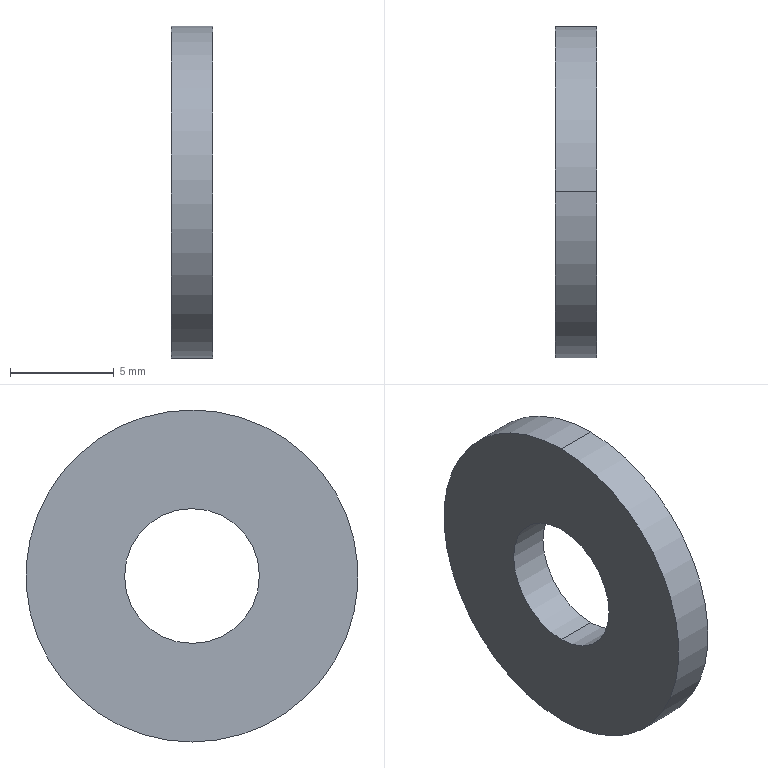Component | SolidWorks | ClampingArm2-1_A73-1 | 1 solid | 6 faces | box 2 x 16 x 16 mm | volume 336 mm3 | cylinder 4 | plane 2 | commonest cylinder face diameters 6.5 x2 16 x2 | material S45C
build123d program:
from build123d import *

# Parameters (mm, degrees)
SKETCH1_R           = 8
SKETCH1_R_2         = 3.25
BOSS_EXTRUDE1_DEPTH = 1


with BuildPart() as part:
    # Sketch1 → Boss-Extrude1 (new, symmetric)
    with BuildSketch(Plane(origin=(0, 0, 0), x_dir=(0, 0, -1), z_dir=(1, 0, 0))):
        Circle(SKETCH1_R)
        Circle(SKETCH1_R_2, mode=Mode.SUBTRACT)
    extrude(amount=BOSS_EXTRUDE1_DEPTH, both=True)


solid = part.part

# Placed as in the assembly
solid = solid.moved(Location((-51.551, 66.036, -52.5), (0, 0, 0)))
STEP:
#1=COLOUR_RGB('',0.7922,0.8196,0.9333);
#2=FILL_AREA_STYLE_COLOUR('',#1);
#3=FILL_AREA_STYLE('',(#2));
#4=SURFACE_STYLE_FILL_AREA(#3);
#5=SURFACE_SIDE_STYLE('',(#4));
#6=SURFACE_STYLE_USAGE(.BOTH.,#5);
#7=PRESENTATION_STYLE_ASSIGNMENT((#6));
#8=CARTESIAN_POINT('',(-1.99,2.6,-1.939));
#9=VERTEX_POINT('',#8);
#10=CARTESIAN_POINT('',(-1.99,2.6,-2.195));
#11=VERTEX_POINT('',#10);
#12=CARTESIAN_POINT('',(-1.99,2.6,-2.067));
#13=DIRECTION('',(1.,0.,-0.));
#14=DIRECTION('',(0.,-0.0003333,-1.));
#15=AXIS2_PLACEMENT_3D('',#12,#13,#14);
#16=CIRCLE('',#15,0.128);
#17=EDGE_CURVE('',#9,#11,#16,.T.);
#18=ORIENTED_EDGE('',*,*,#17,.T.);
#19=CARTESIAN_POINT('',(-2.069,2.6,-2.195));
#20=VERTEX_POINT('',#19);
#21=CARTESIAN_POINT('',(-1.99,2.6,-2.195));
#22=DIRECTION('',(-1.,-0.,0.));
#23=VECTOR('',#22,39.37);
#24=LINE('',#21,#23);
#25=EDGE_CURVE('',#11,#20,#24,.T.);
#26=ORIENTED_EDGE('',*,*,#25,.T.);
#27=CARTESIAN_POINT('',(-2.069,2.6,-1.939));
#28=VERTEX_POINT('',#27);
#29=CARTESIAN_POINT('',(-2.069,2.6,-2.067));
#30=DIRECTION('',(1.,0.,-0.));
#31=DIRECTION('',(0.,-0.0003333,-1.));
#32=AXIS2_PLACEMENT_3D('',#29,#30,#31);
#33=CIRCLE('',#32,0.128);
#34=EDGE_CURVE('',#28,#20,#33,.T.);
#35=ORIENTED_EDGE('',*,*,#34,.F.);
#36=CARTESIAN_POINT('',(-1.99,2.6,-1.939));
#37=DIRECTION('',(-1.,-0.,0.));
#38=VECTOR('',#37,39.37);
#39=LINE('',#36,#38);
#40=EDGE_CURVE('',#9,#28,#39,.T.);
#41=ORIENTED_EDGE('',*,*,#40,.F.);
#42=EDGE_LOOP('',(#18,#26,#35,#41));
#43=FACE_OUTER_BOUND('',#42,.T.);
#44=CARTESIAN_POINT('',(-1.99,2.6,-2.067));
#45=DIRECTION('',(-1.,-0.,0.));
#46=DIRECTION('',(0.,0.0003333,1.));
#47=AXIS2_PLACEMENT_3D('',#44,#45,#46);
#48=CYLINDRICAL_SURFACE('',#47,0.128);
#49=ADVANCED_FACE('',(#43),#48,.F.);
#50=CARTESIAN_POINT('',(-1.99,2.6,-2.382));
#51=VERTEX_POINT('',#50);
#52=CARTESIAN_POINT('',(-1.99,2.6,-1.752));
#53=VERTEX_POINT('',#52);
#54=CARTESIAN_POINT('',(-1.99,2.6,-2.067));
#55=DIRECTION('',(1.,0.,-0.));
#56=DIRECTION('',(0.,-0.0003333,-1.));
#57=AXIS2_PLACEMENT_3D('',#54,#55,#56);
#58=CIRCLE('',#57,0.315);
#59=EDGE_CURVE('',#51,#53,#58,.T.);
#60=ORIENTED_EDGE('',*,*,#59,.F.);
#61=CARTESIAN_POINT('',(-2.069,2.6,-2.382));
#62=VERTEX_POINT('',#61);
#63=CARTESIAN_POINT('',(-1.99,2.6,-2.382));
#64=DIRECTION('',(-1.,-0.,0.));
#65=VECTOR('',#64,39.37);
#66=LINE('',#63,#65);
#67=EDGE_CURVE('',#51,#62,#66,.T.);
#68=ORIENTED_EDGE('',*,*,#67,.T.);
#69=CARTESIAN_POINT('',(-2.069,2.6,-1.752));
#70=VERTEX_POINT('',#69);
#71=CARTESIAN_POINT('',(-2.069,2.6,-2.067));
#72=DIRECTION('',(1.,0.,-0.));
#73=DIRECTION('',(0.,-0.0003333,-1.));
#74=AXIS2_PLACEMENT_3D('',#71,#72,#73);
#75=CIRCLE('',#74,0.315);
#76=EDGE_CURVE('',#62,#70,#75,.T.);
#77=ORIENTED_EDGE('',*,*,#76,.T.);
#78=CARTESIAN_POINT('',(-1.99,2.6,-1.752));
#79=DIRECTION('',(-1.,-0.,0.));
#80=VECTOR('',#79,39.37);
#81=LINE('',#78,#80);
#82=EDGE_CURVE('',#53,#70,#81,.T.);
#83=ORIENTED_EDGE('',*,*,#82,.F.);
#84=EDGE_LOOP('',(#60,#68,#77,#83));
#85=FACE_OUTER_BOUND('',#84,.T.);
#86=CARTESIAN_POINT('',(-1.99,2.6,-2.067));
#87=DIRECTION('',(-1.,-0.,0.));
#88=DIRECTION('',(0.,0.0003333,1.));
#89=AXIS2_PLACEMENT_3D('',#86,#87,#88);
#90=CYLINDRICAL_SURFACE('',#89,0.315);
#91=ADVANCED_FACE('',(#85),#90,.T.);
#92=CARTESIAN_POINT('',(-1.99,2.6,-2.067));
#93=DIRECTION('',(1.,0.,-0.));
#94=DIRECTION('',(0.,-0.0003333,-1.));
#95=AXIS2_PLACEMENT_3D('',#92,#93,#94);
#96=CIRCLE('',#95,0.315);
#97=EDGE_CURVE('',#53,#51,#96,.T.);
#98=ORIENTED_EDGE('',*,*,#97,.T.);
#99=ORIENTED_EDGE('',*,*,#59,.T.);
#100=EDGE_LOOP('',(#98,#99));
#101=FACE_OUTER_BOUND('',#100,.T.);
#102=ORIENTED_EDGE('',*,*,#17,.F.);
#103=CARTESIAN_POINT('',(-1.99,2.6,-2.067));
#104=DIRECTION('',(1.,0.,-0.));
#105=DIRECTION('',(0.,-0.0003333,-1.));
#106=AXIS2_PLACEMENT_3D('',#103,#104,#105);
#107=CIRCLE('',#106,0.128);
#108=EDGE_CURVE('',#11,#9,#107,.T.);
#109=ORIENTED_EDGE('',*,*,#108,.F.);
#110=EDGE_LOOP('',(#102,#109));
#111=FACE_BOUND('',#110,.T.);
#112=CARTESIAN_POINT('',(-1.99,2.6,-2.067));
#113=DIRECTION('',(1.,0.,-0.));
#114=DIRECTION('',(-0.,-0.0003333,-1.));
#115=AXIS2_PLACEMENT_3D('',#112,#113,#114);
#116=PLANE('',#115);
#117=ADVANCED_FACE('',(#101,#111),#116,.T.);
#118=CARTESIAN_POINT('',(-2.069,2.6,-2.067));
#119=DIRECTION('',(1.,0.,-0.));
#120=DIRECTION('',(0.,-0.0003333,-1.));
#121=AXIS2_PLACEMENT_3D('',#118,#119,#120);
#122=CIRCLE('',#121,0.315);
#123=EDGE_CURVE('',#70,#62,#122,.T.);
#124=ORIENTED_EDGE('',*,*,#123,.F.);
#125=ORIENTED_EDGE('',*,*,#76,.F.);
#126=EDGE_LOOP('',(#124,#125));
#127=FACE_OUTER_BOUND('',#126,.T.);
#128=ORIENTED_EDGE('',*,*,#34,.T.);
#129=CARTESIAN_POINT('',(-2.069,2.6,-2.067));
#130=DIRECTION('',(1.,0.,-0.));
#131=DIRECTION('',(0.,-0.0003333,-1.));
#132=AXIS2_PLACEMENT_3D('',#129,#130,#131);
#133=CIRCLE('',#132,0.128);
#134=EDGE_CURVE('',#20,#28,#133,.T.);
#135=ORIENTED_EDGE('',*,*,#134,.T.);
#136=EDGE_LOOP('',(#128,#135));
#137=FACE_BOUND('',#136,.T.);
#138=CARTESIAN_POINT('',(-2.069,2.6,-2.067));
#139=DIRECTION('',(1.,0.,-0.));
#140=DIRECTION('',(-0.,-0.0003333,-1.));
#141=AXIS2_PLACEMENT_3D('',#138,#139,#140);
#142=PLANE('',#141);
#143=ADVANCED_FACE('',(#127,#137),#142,.F.);
#144=ORIENTED_EDGE('',*,*,#67,.F.);
#145=ORIENTED_EDGE('',*,*,#97,.F.);
#146=ORIENTED_EDGE('',*,*,#82,.T.);
#147=ORIENTED_EDGE('',*,*,#123,.T.);
#148=EDGE_LOOP('',(#144,#145,#146,#147));
#149=FACE_OUTER_BOUND('',#148,.T.);
#150=CARTESIAN_POINT('',(-1.99,2.6,-2.067));
#151=DIRECTION('',(-1.,-0.,0.));
#152=DIRECTION('',(0.,0.0003333,1.));
#153=AXIS2_PLACEMENT_3D('',#150,#151,#152);
#154=CYLINDRICAL_SURFACE('',#153,0.315);
#155=ADVANCED_FACE('',(#149),#154,.T.);
#156=ORIENTED_EDGE('',*,*,#25,.F.);
#157=ORIENTED_EDGE('',*,*,#108,.T.);
#158=ORIENTED_EDGE('',*,*,#40,.T.);
#159=ORIENTED_EDGE('',*,*,#134,.F.);
#160=EDGE_LOOP('',(#156,#157,#158,#159));
#161=FACE_OUTER_BOUND('',#160,.T.);
#162=CARTESIAN_POINT('',(-1.99,2.6,-2.067));
#163=DIRECTION('',(-1.,-0.,0.));
#164=DIRECTION('',(0.,0.0003333,1.));
#165=AXIS2_PLACEMENT_3D('',#162,#163,#164);
#166=CYLINDRICAL_SURFACE('',#165,0.128);
#167=ADVANCED_FACE('',(#161),#166,.F.);
#168=CLOSED_SHELL('',(#49,#91,#117,#143,#155,#167));
#169=MANIFOLD_SOLID_BREP('',#168);
#170=STYLED_ITEM('',(#7),#169);
#171=(LENGTH_UNIT()NAMED_UNIT(*)SI_UNIT($,.METRE.));
#172=LENGTH_MEASURE_WITH_UNIT(LENGTH_MEASURE(0.0254),#171);
#173=DIMENSIONAL_EXPONENTS(1.,0.,0.,0.,0.,0.,0.);
#174=(CONVERSION_BASED_UNIT('',#172)LENGTH_UNIT()NAMED_UNIT(#173));
#175=UNCERTAINTY_MEASURE_WITH_UNIT(LENGTH_MEASURE(0.00001),#174,'','');
#176=(NAMED_UNIT(*)PLANE_ANGLE_UNIT()SI_UNIT($,.RADIAN.));
#177=(NAMED_UNIT(*)SI_UNIT($,.STERADIAN.)SOLID_ANGLE_UNIT());
#178=(GEOMETRIC_REPRESENTATION_CONTEXT(3)GLOBAL_UNCERTAINTY_ASSIGNED_CONTEXT((#175))GLOBAL_UNIT_ASSIGNED_CONTEXT((#174,#176,#177))REPRESENTATION_CONTEXT('',''));
#179=MECHANICAL_DESIGN_GEOMETRIC_PRESENTATION_REPRESENTATION('',(#170),#178);
#180=PRESENTATION_LAYER_ASSIGNMENT('','',(#170));
#181=CARTESIAN_POINT('',(0.,0.,0.));
#182=DIRECTION('',(0.,0.,1.));
#183=DIRECTION('',(1.,0.,0.));
#184=AXIS2_PLACEMENT_3D('',#181,#182,#183);
#185=(LENGTH_UNIT()NAMED_UNIT(*)SI_UNIT($,.METRE.));
#186=LENGTH_MEASURE_WITH_UNIT(LENGTH_MEASURE(0.0254),#185);
#187=DIMENSIONAL_EXPONENTS(1.,0.,0.,0.,0.,0.,0.);
#188=(CONVERSION_BASED_UNIT('',#186)LENGTH_UNIT()NAMED_UNIT(#187));
#189=UNCERTAINTY_MEASURE_WITH_UNIT(LENGTH_MEASURE(0.00001),#188,'','');
#190=(NAMED_UNIT(*)PLANE_ANGLE_UNIT()SI_UNIT($,.RADIAN.));
#191=(NAMED_UNIT(*)SI_UNIT($,.STERADIAN.)SOLID_ANGLE_UNIT());
#192=(GEOMETRIC_REPRESENTATION_CONTEXT(3)GLOBAL_UNCERTAINTY_ASSIGNED_CONTEXT((#189))GLOBAL_UNIT_ASSIGNED_CONTEXT((#188,#190,#191))REPRESENTATION_CONTEXT('',''));
#193=ADVANCED_BREP_SHAPE_REPRESENTATION('',(#169,#184),#192);